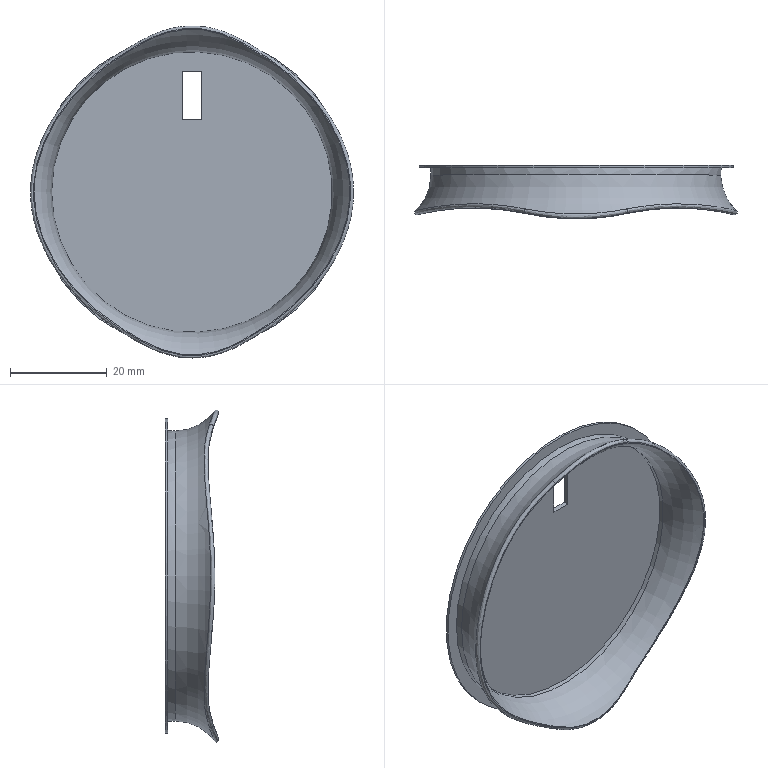Component | NX | FRUIT_TRAY | 1 solid | 20 faces | volume 4811 mm3 | plane 7 | cylinder 7 | spline 4 | torus 2 | commonest cylinder face diameters 100 x4 65 x1 60 x1 58 x1